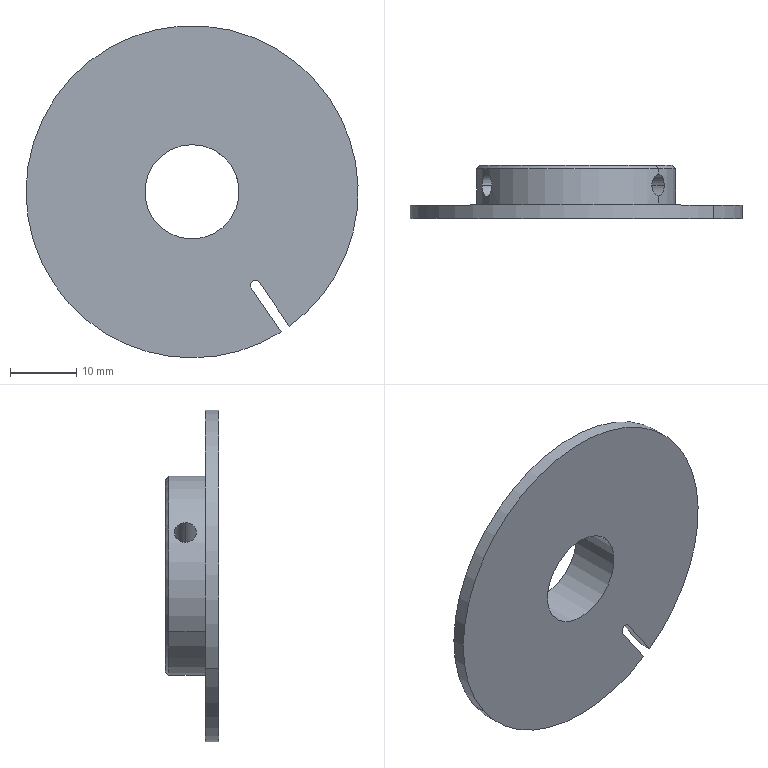Component | SolidWorks | H2020022-0437-1-2 | 1 solid | 19 faces | box 50 x 8 x 50 mm | volume 6728 mm3 | cylinder 12 | plane 5 | cone 2 | commonest cylinder face diameters 3.3 x4 50 x3 14.2 x2 30 x2 1.5 x1 | material 45#Steel
build123d program:
from build123d import *

# Parameters (mm, degrees)
SKETCH1_R           = 15
SKETCH1_R_2         = 7.1
BOSS_EXTRUDE1_DEPTH = 8
SKETCH3_W           = 1.65
SKETCH3_H           = 15
CIRPATTERN1_COUNT   = 2
CIRPATTERN1_ANGLE   = 120
CHAMFER2_SIZE       = 0.5
BOSS_EXTRUDE2_START = -2
SKETCH6_R           = 25
SKETCH6_R_2         = 15
BOSS_EXTRUDE2_DEPTH = 2
CUT_EXTRUDE1_DEPTH  = 37.249


with BuildPart() as part:
    # Sketch1 → Boss-Extrude1 (new body)
    with BuildSketch(Plane(origin=(0, 0, 0), x_dir=(1, 0, 0), z_dir=(0, 1, 0))):
        with Locations(Location((0, 0, 0), (0, 0, 270))):
            Circle(SKETCH1_R)
        with Locations(Location((0, 0, 0), (0, 0, 270))):
            Circle(SKETCH1_R_2, mode=Mode.SUBTRACT)
    extrude(amount=BOSS_EXTRUDE1_DEPTH)

    # Sketch3 → M4 Tapped Hole2 (revolve, cut)
    with BuildSketch(Plane(origin=(0, 3, 0), x_dir=(0, 1, 0), z_dir=(1, 0, 0))):
        with Locations((0.825, 7.5)):
            Rectangle(SKETCH3_W, SKETCH3_H)
    m4_tapped_hole2 = revolve(axis=Axis((0, 3, -6.35), (0, 0, 1)), mode=Mode.SUBTRACT)

    # CirPattern1: M4 Tapped Hole2 ×2 about axis
    cirpattern1_axis = Axis((0, 8, 0), (0, 1, 0))
    for i in range(1, CIRPATTERN1_COUNT):
        add(m4_tapped_hole2.rotate(cirpattern1_axis, i * CIRPATTERN1_ANGLE / (CIRPATTERN1_COUNT - 1)), mode=Mode.SUBTRACT)

    # Chamfer2
    chamfer2_edges = [part.edges().sort_by_distance(p)[0] for p in [
        (0, 0, -15),
    ]]
    chamfer(chamfer2_edges, length=CHAMFER2_SIZE)

    # Sketch6 → Boss-Extrude2 (add)
    with BuildSketch(Plane(origin=(0, 8, 0), x_dir=(1, 0, 0), z_dir=(0, 1, 0)).offset(BOSS_EXTRUDE2_START)):
        with Locations(Location((0, 0, 0), (0, 0, 270))):
            Circle(SKETCH6_R)
        with Locations(Location((0, 0, 0), (0, 0, 270))):
            Circle(SKETCH6_R_2, mode=Mode.SUBTRACT)
    extrude(amount=BOSS_EXTRUDE2_DEPTH)

    # Sketch7 → Cut-Extrude1 (cut, through all)
    with BuildSketch(Plane(origin=(0, 8, 0), x_dir=(1, 0, 0), z_dir=(0, 1, 0))):
        with BuildLine():
            Line((-25, 0.75), (-17, 0.75))
            ThreePointArc((-17, 0.75), (-16.25, 0), (-17, -0.75))
            Line((-17, -0.75), (-25, -0.75))
            ThreePointArc((-25, -0.75), (-25.75, 0), (-25, 0.75))
        make_face()
    extrude(amount=-CUT_EXTRUDE1_DEPTH, mode=Mode.SUBTRACT)


solid = part.part

# Placed as in the assembly
solid = solid.moved(Location((-30.964, 61.013, 280.197), (0, 55.863, 180)))
STEP:
#1=COLOUR_RGB('',0.7922,0.8196,0.9333);
#2=FILL_AREA_STYLE_COLOUR('',#1);
#3=FILL_AREA_STYLE('',(#2));
#4=SURFACE_STYLE_FILL_AREA(#3);
#5=SURFACE_SIDE_STYLE('',(#4));
#6=SURFACE_STYLE_USAGE(.BOTH.,#5);
#7=PRESENTATION_STYLE_ASSIGNMENT((#6));
#8=CARTESIAN_POINT('',(-0.4044,2.166,11.584));
#9=VERTEX_POINT('',#8);
#10=CARTESIAN_POINT('',(-2.034,2.166,10.479));
#11=VERTEX_POINT('',#10);
#12=CARTESIAN_POINT('',(-1.219,2.166,11.031));
#13=DIRECTION('',(0.,-1.,0.));
#14=DIRECTION('',(0.8277,0.,0.5612));
#15=AXIS2_PLACEMENT_3D('',#12,#13,#14);
#16=CIRCLE('',#15,0.9843);
#17=EDGE_CURVE('',#9,#11,#16,.T.);
#18=ORIENTED_EDGE('',*,*,#17,.T.);
#19=CARTESIAN_POINT('',(-2.034,2.087,10.479));
#20=VERTEX_POINT('',#19);
#21=CARTESIAN_POINT('',(-2.034,2.166,10.479));
#22=DIRECTION('',(0.,-1.,0.));
#23=VECTOR('',#22,39.37);
#24=LINE('',#21,#23);
#25=EDGE_CURVE('',#11,#20,#24,.T.);
#26=ORIENTED_EDGE('',*,*,#25,.T.);
#27=CARTESIAN_POINT('',(-0.4044,2.087,11.584));
#28=VERTEX_POINT('',#27);
#29=CARTESIAN_POINT('',(-1.219,2.087,11.031));
#30=DIRECTION('',(0.,-1.,0.));
#31=DIRECTION('',(0.8277,0.,0.5612));
#32=AXIS2_PLACEMENT_3D('',#29,#30,#31);
#33=CIRCLE('',#32,0.9843);
#34=EDGE_CURVE('',#28,#20,#33,.T.);
#35=ORIENTED_EDGE('',*,*,#34,.F.);
#36=CARTESIAN_POINT('',(-0.4044,2.166,11.584));
#37=DIRECTION('',(0.,-1.,0.));
#38=VECTOR('',#37,39.37);
#39=LINE('',#36,#38);
#40=EDGE_CURVE('',#9,#28,#39,.T.);
#41=ORIENTED_EDGE('',*,*,#40,.F.);
#42=EDGE_LOOP('',(#18,#26,#35,#41));
#43=FACE_OUTER_BOUND('',#42,.T.);
#44=CARTESIAN_POINT('',(-1.219,2.166,11.031));
#45=DIRECTION('',(0.,-1.,0.));
#46=DIRECTION('',(0.8277,0.,0.5612));
#47=AXIS2_PLACEMENT_3D('',#44,#45,#46);
#48=CYLINDRICAL_SURFACE('',#47,0.9843);
#49=ADVANCED_FACE('',(#43),#48,.T.);
#50=CARTESIAN_POINT('',(-0.6425,2.166,10.234));
#51=VERTEX_POINT('',#50);
#52=CARTESIAN_POINT('',(-1.219,2.166,11.031));
#53=DIRECTION('',(0.,-1.,0.));
#54=DIRECTION('',(0.8277,0.,0.5612));
#55=AXIS2_PLACEMENT_3D('',#52,#53,#54);
#56=CIRCLE('',#55,0.9843);
#57=EDGE_CURVE('',#51,#9,#56,.T.);
#58=ORIENTED_EDGE('',*,*,#57,.T.);
#59=ORIENTED_EDGE('',*,*,#40,.T.);
#60=CARTESIAN_POINT('',(-0.6425,2.087,10.234));
#61=VERTEX_POINT('',#60);
#62=CARTESIAN_POINT('',(-1.219,2.087,11.031));
#63=DIRECTION('',(0.,-1.,0.));
#64=DIRECTION('',(0.8277,0.,0.5612));
#65=AXIS2_PLACEMENT_3D('',#62,#63,#64);
#66=CIRCLE('',#65,0.9843);
#67=EDGE_CURVE('',#61,#28,#66,.T.);
#68=ORIENTED_EDGE('',*,*,#67,.F.);
#69=CARTESIAN_POINT('',(-0.6425,2.166,10.234));
#70=DIRECTION('',(0.,-1.,0.));
#71=VECTOR('',#70,39.37);
#72=LINE('',#69,#71);
#73=EDGE_CURVE('',#51,#61,#72,.T.);
#74=ORIENTED_EDGE('',*,*,#73,.F.);
#75=EDGE_LOOP('',(#58,#59,#68,#74));
#76=FACE_OUTER_BOUND('',#75,.T.);
#77=CARTESIAN_POINT('',(-1.219,2.166,11.031));
#78=DIRECTION('',(0.,-1.,0.));
#79=DIRECTION('',(0.8277,0.,0.5612));
#80=AXIS2_PLACEMENT_3D('',#77,#78,#79);
#81=CYLINDRICAL_SURFACE('',#80,0.9843);
#82=ADVANCED_FACE('',(#76),#81,.T.);
#83=CARTESIAN_POINT('',(-1.692,2.402,10.711));
#84=VERTEX_POINT('',#83);
#85=CARTESIAN_POINT('',(-0.7466,2.402,11.352));
#86=VERTEX_POINT('',#85);
#87=CARTESIAN_POINT('',(-1.219,2.402,11.031));
#88=DIRECTION('',(0.,1.,0.));
#89=DIRECTION('',(0.8277,0.,0.5612));
#90=AXIS2_PLACEMENT_3D('',#87,#88,#89);
#91=CIRCLE('',#90,0.5709);
#92=EDGE_CURVE('',#84,#86,#91,.T.);
#93=ORIENTED_EDGE('',*,*,#92,.F.);
#94=CARTESIAN_POINT('',(-1.708,2.382,10.7));
#95=VERTEX_POINT('',#94);
#96=CARTESIAN_POINT('',(-1.708,2.382,10.7));
#97=DIRECTION('',(-0.5853,-0.7071,-0.3968));
#98=VECTOR('',#97,39.37);
#99=LINE('',#96,#98);
#100=EDGE_CURVE('',#84,#95,#99,.T.);
#101=ORIENTED_EDGE('',*,*,#100,.T.);
#102=CARTESIAN_POINT('',(-0.7303,2.382,11.363));
#103=VERTEX_POINT('',#102);
#104=CARTESIAN_POINT('',(-1.219,2.382,11.031));
#105=DIRECTION('',(0.,-1.,0.));
#106=DIRECTION('',(0.8277,0.,0.5612));
#107=AXIS2_PLACEMENT_3D('',#104,#105,#106);
#108=CIRCLE('',#107,0.5906);
#109=EDGE_CURVE('',#103,#95,#108,.T.);
#110=ORIENTED_EDGE('',*,*,#109,.F.);
#111=CARTESIAN_POINT('',(-0.7303,2.382,11.363));
#112=DIRECTION('',(0.5853,-0.7071,0.3968));
#113=VECTOR('',#112,39.37);
#114=LINE('',#111,#113);
#115=EDGE_CURVE('',#86,#103,#114,.T.);
#116=ORIENTED_EDGE('',*,*,#115,.F.);
#117=EDGE_LOOP('',(#93,#101,#110,#116));
#118=FACE_OUTER_BOUND('',#117,.T.);
#119=CARTESIAN_POINT('',(-1.219,2.382,11.031));
#120=DIRECTION('',(0.,-1.,0.));
#121=DIRECTION('',(0.8277,0.,0.5612));
#122=AXIS2_PLACEMENT_3D('',#119,#120,#121);
#123=CONICAL_SURFACE('',#122,0.5906,0.7854);
#124=ADVANCED_FACE('',(#118),#123,.T.);
#125=CARTESIAN_POINT('',(-1.776,2.284,11.229));
#126=VERTEX_POINT('',#125);
#127=CARTESIAN_POINT('',(-1.719,2.284,11.346));
#128=VERTEX_POINT('',#127);
#129=CARTESIAN_POINT('',(-1.776,2.284,11.229));
#130=CARTESIAN_POINT('',(-1.776,2.292,11.229));
#131=CARTESIAN_POINT('',(-1.775,2.301,11.231));
#132=CARTESIAN_POINT('',(-1.773,2.317,11.237));
#133=CARTESIAN_POINT('',(-1.771,2.324,11.241));
#134=CARTESIAN_POINT('',(-1.768,2.333,11.25));
#135=CARTESIAN_POINT('',(-1.767,2.336,11.253));
#136=CARTESIAN_POINT('',(-1.764,2.34,11.259));
#137=CARTESIAN_POINT('',(-1.762,2.342,11.263));
#138=CARTESIAN_POINT('',(-1.759,2.346,11.27));
#139=CARTESIAN_POINT('',(-1.758,2.347,11.274));
#140=CARTESIAN_POINT('',(-1.754,2.348,11.281));
#141=CARTESIAN_POINT('',(-1.752,2.349,11.285));
#142=CARTESIAN_POINT('',(-1.749,2.349,11.293));
#143=CARTESIAN_POINT('',(-1.747,2.349,11.297));
#144=CARTESIAN_POINT('',(-1.743,2.347,11.304));
#145=CARTESIAN_POINT('',(-1.741,2.346,11.308));
#146=CARTESIAN_POINT('',(-1.737,2.342,11.315));
#147=CARTESIAN_POINT('',(-1.735,2.34,11.318));
#148=CARTESIAN_POINT('',(-1.732,2.336,11.324));
#149=CARTESIAN_POINT('',(-1.73,2.333,11.327));
#150=CARTESIAN_POINT('',(-1.726,2.324,11.335));
#151=CARTESIAN_POINT('',(-1.723,2.317,11.339));
#152=CARTESIAN_POINT('',(-1.72,2.301,11.344));
#153=CARTESIAN_POINT('',(-1.719,2.293,11.346));
#154=CARTESIAN_POINT('',(-1.719,2.284,11.346));
#155=B_SPLINE_CURVE_WITH_KNOTS('',3,(#129,#130,#131,#132,#133,#134,#135,#136,#137,#138,#139,#140,#141,#142,#143,#144,#145,#146,#147,#148,#149,#150,#151,#152,#153,#154),.UNSPECIFIED.,.F.,.F.,(4,2,2,2,2,2,2,2,2,2,2,2,4),(0.005163,0.005808,0.006453,0.006775,0.007098,0.007421,0.007743,0.008066,0.008388,0.008711,0.009034,0.009679,0.01032),.UNSPECIFIED.);
#156=EDGE_CURVE('',#126,#128,#155,.T.);
#157=ORIENTED_EDGE('',*,*,#156,.F.);
#158=CARTESIAN_POINT('',(-1.492,2.284,11.092));
#159=VERTEX_POINT('',#158);
#160=CARTESIAN_POINT('',(-1.247,2.284,10.973));
#161=DIRECTION('',(0.8998,0.,-0.4362));
#162=VECTOR('',#161,39.37);
#163=LINE('',#160,#162);
#164=EDGE_CURVE('',#126,#159,#163,.T.);
#165=ORIENTED_EDGE('',*,*,#164,.T.);
#166=CARTESIAN_POINT('',(-1.435,2.284,11.208));
#167=VERTEX_POINT('',#166);
#168=CARTESIAN_POINT('',(-1.492,2.284,11.092));
#169=CARTESIAN_POINT('',(-1.492,2.292,11.092));
#170=CARTESIAN_POINT('',(-1.492,2.301,11.093));
#171=CARTESIAN_POINT('',(-1.491,2.313,11.098));
#172=CARTESIAN_POINT('',(-1.49,2.317,11.1));
#173=CARTESIAN_POINT('',(-1.489,2.324,11.105));
#174=CARTESIAN_POINT('',(-1.488,2.327,11.107));
#175=CARTESIAN_POINT('',(-1.486,2.333,11.113));
#176=CARTESIAN_POINT('',(-1.485,2.336,11.116));
#177=CARTESIAN_POINT('',(-1.483,2.34,11.123));
#178=CARTESIAN_POINT('',(-1.482,2.342,11.127));
#179=CARTESIAN_POINT('',(-1.478,2.347,11.138));
#180=CARTESIAN_POINT('',(-1.474,2.349,11.146));
#181=CARTESIAN_POINT('',(-1.469,2.349,11.157));
#182=CARTESIAN_POINT('',(-1.467,2.349,11.161));
#183=CARTESIAN_POINT('',(-1.463,2.347,11.168));
#184=CARTESIAN_POINT('',(-1.461,2.346,11.172));
#185=CARTESIAN_POINT('',(-1.455,2.341,11.182));
#186=CARTESIAN_POINT('',(-1.451,2.336,11.188));
#187=CARTESIAN_POINT('',(-1.444,2.324,11.198));
#188=CARTESIAN_POINT('',(-1.441,2.317,11.202));
#189=CARTESIAN_POINT('',(-1.438,2.305,11.206));
#190=CARTESIAN_POINT('',(-1.437,2.301,11.207));
#191=CARTESIAN_POINT('',(-1.436,2.293,11.208));
#192=CARTESIAN_POINT('',(-1.435,2.288,11.208));
#193=CARTESIAN_POINT('',(-1.435,2.284,11.208));
#194=B_SPLINE_CURVE_WITH_KNOTS('',3,(#168,#169,#170,#171,#172,#173,#174,#175,#176,#177,#178,#179,#180,#181,#182,#183,#184,#185,#186,#187,#188,#189,#190,#191,#192,#193),.UNSPECIFIED.,.F.,.F.,(4,2,2,2,2,2,2,2,2,2,2,2,4),(0.005176,0.005823,0.006147,0.00647,0.006794,0.007117,0.007764,0.008087,0.008411,0.009058,0.009704,0.01003,0.01035),.UNSPECIFIED.);
#195=EDGE_CURVE('',#159,#167,#194,.T.);
#196=ORIENTED_EDGE('',*,*,#195,.T.);
#197=CARTESIAN_POINT('',(-1.191,2.284,11.09));
#198=DIRECTION('',(0.8998,0.,-0.4362));
#199=VECTOR('',#198,39.37);
#200=LINE('',#197,#199);
#201=EDGE_CURVE('',#128,#167,#200,.T.);
#202=ORIENTED_EDGE('',*,*,#201,.F.);
#203=EDGE_LOOP('',(#157,#165,#196,#202));
#204=FACE_OUTER_BOUND('',#203,.T.);
#205=CARTESIAN_POINT('',(-1.219,2.284,11.031));
#206=DIRECTION('',(0.8998,0.,-0.4362));
#207=DIRECTION('',(0.4362,0.,0.8998));
#208=AXIS2_PLACEMENT_3D('',#205,#206,#207);
#209=CYLINDRICAL_SURFACE('',#208,0.06496);
#210=ADVANCED_FACE('',(#204),#209,.F.);
#211=CARTESIAN_POINT('',(-0.7697,2.284,11.415));
#212=VERTEX_POINT('',#211);
#213=CARTESIAN_POINT('',(-0.7303,2.349,11.363));
#214=VERTEX_POINT('',#213);
#215=CARTESIAN_POINT('',(-0.7697,2.284,11.415));
#216=CARTESIAN_POINT('',(-0.7697,2.288,11.415));
#217=CARTESIAN_POINT('',(-0.7694,2.292,11.414));
#218=CARTESIAN_POINT('',(-0.7683,2.301,11.413));
#219=CARTESIAN_POINT('',(-0.7675,2.305,11.412));
#220=CARTESIAN_POINT('',(-0.7654,2.313,11.409));
#221=CARTESIAN_POINT('',(-0.7641,2.316,11.408));
#222=CARTESIAN_POINT('',(-0.7611,2.324,11.404));
#223=CARTESIAN_POINT('',(-0.7594,2.327,11.402));
#224=CARTESIAN_POINT('',(-0.7538,2.336,11.395));
#225=CARTESIAN_POINT('',(-0.7493,2.341,11.389));
#226=CARTESIAN_POINT('',(-0.74,2.347,11.377));
#227=CARTESIAN_POINT('',(-0.7351,2.349,11.37));
#228=CARTESIAN_POINT('',(-0.7303,2.349,11.363));
#229=B_SPLINE_CURVE_WITH_KNOTS('',3,(#215,#216,#217,#218,#219,#220,#221,#222,#223,#224,#225,#226,#227,#228),.UNSPECIFIED.,.F.,.F.,(4,2,2,2,2,2,4),(0.007744,0.008067,0.008389,0.008712,0.009034,0.009679,0.01032),.UNSPECIFIED.);
#230=EDGE_CURVE('',#212,#214,#229,.T.);
#231=ORIENTED_EDGE('',*,*,#230,.F.);
#232=CARTESIAN_POINT('',(-1.03,2.284,11.238));
#233=VERTEX_POINT('',#232);
#234=CARTESIAN_POINT('',(-1.256,2.284,11.085));
#235=DIRECTION('',(-0.8277,0.,-0.5612));
#236=VECTOR('',#235,39.37);
#237=LINE('',#234,#236);
#238=EDGE_CURVE('',#212,#233,#237,.T.);
#239=ORIENTED_EDGE('',*,*,#238,.T.);
#240=CARTESIAN_POINT('',(-0.9877,2.349,11.188));
#241=VERTEX_POINT('',#240);
#242=CARTESIAN_POINT('',(-1.03,2.284,11.238));
#243=CARTESIAN_POINT('',(-1.03,2.292,11.238));
#244=CARTESIAN_POINT('',(-1.029,2.301,11.237));
#245=CARTESIAN_POINT('',(-1.026,2.313,11.233));
#246=CARTESIAN_POINT('',(-1.024,2.317,11.232));
#247=CARTESIAN_POINT('',(-1.021,2.324,11.228));
#248=CARTESIAN_POINT('',(-1.019,2.327,11.226));
#249=CARTESIAN_POINT('',(-1.015,2.333,11.222));
#250=CARTESIAN_POINT('',(-1.012,2.336,11.219));
#251=CARTESIAN_POINT('',(-1.008,2.34,11.214));
#252=CARTESIAN_POINT('',(-1.005,2.342,11.211));
#253=CARTESIAN_POINT('',(-0.9976,2.347,11.202));
#254=CARTESIAN_POINT('',(-0.9925,2.349,11.195));
#255=CARTESIAN_POINT('',(-0.9877,2.349,11.188));
#256=B_SPLINE_CURVE_WITH_KNOTS('',3,(#242,#243,#244,#245,#246,#247,#248,#249,#250,#251,#252,#253,#254,#255),.UNSPECIFIED.,.F.,.F.,(4,2,2,2,2,2,4),(0.005176,0.005823,0.006147,0.00647,0.006794,0.007117,0.007764),.UNSPECIFIED.);
#257=EDGE_CURVE('',#233,#241,#256,.T.);
#258=ORIENTED_EDGE('',*,*,#257,.T.);
#259=CARTESIAN_POINT('',(-0.9576,2.284,11.13));
#260=VERTEX_POINT('',#259);
#261=CARTESIAN_POINT('',(-0.9877,2.349,11.188));
#262=CARTESIAN_POINT('',(-0.9853,2.349,11.185));
#263=CARTESIAN_POINT('',(-0.983,2.349,11.181));
#264=CARTESIAN_POINT('',(-0.9786,2.347,11.174));
#265=CARTESIAN_POINT('',(-0.9766,2.346,11.17));
#266=CARTESIAN_POINT('',(-0.9708,2.341,11.16));
#267=CARTESIAN_POINT('',(-0.9676,2.336,11.154));
#268=CARTESIAN_POINT('',(-0.9625,2.324,11.143));
#269=CARTESIAN_POINT('',(-0.9607,2.317,11.138));
#270=CARTESIAN_POINT('',(-0.9588,2.305,11.133));
#271=CARTESIAN_POINT('',(-0.9583,2.301,11.132));
#272=CARTESIAN_POINT('',(-0.9577,2.293,11.131));
#273=CARTESIAN_POINT('',(-0.9576,2.288,11.13));
#274=CARTESIAN_POINT('',(-0.9576,2.284,11.13));
#275=B_SPLINE_CURVE_WITH_KNOTS('',3,(#261,#262,#263,#264,#265,#266,#267,#268,#269,#270,#271,#272,#273,#274),.UNSPECIFIED.,.F.,.F.,(4,2,2,2,2,2,4),(0.007764,0.008088,0.008411,0.009058,0.009705,0.01003,0.01035),.UNSPECIFIED.);
#276=EDGE_CURVE('',#241,#260,#275,.T.);
#277=ORIENTED_EDGE('',*,*,#276,.T.);
#278=CARTESIAN_POINT('',(-0.6968,2.284,11.307));
#279=VERTEX_POINT('',#278);
#280=CARTESIAN_POINT('',(-1.183,2.284,10.978));
#281=DIRECTION('',(-0.8277,0.,-0.5612));
#282=VECTOR('',#281,39.37);
#283=LINE('',#280,#282);
#284=EDGE_CURVE('',#279,#260,#283,.T.);
#285=ORIENTED_EDGE('',*,*,#284,.F.);
#286=CARTESIAN_POINT('',(-0.7303,2.349,11.363));
#287=CARTESIAN_POINT('',(-0.7279,2.349,11.359));
#288=CARTESIAN_POINT('',(-0.7255,2.349,11.356));
#289=CARTESIAN_POINT('',(-0.721,2.347,11.349));
#290=CARTESIAN_POINT('',(-0.7188,2.346,11.345));
#291=CARTESIAN_POINT('',(-0.7147,2.342,11.339));
#292=CARTESIAN_POINT('',(-0.7127,2.34,11.335));
#293=CARTESIAN_POINT('',(-0.7091,2.336,11.329));
#294=CARTESIAN_POINT('',(-0.7074,2.333,11.326));
#295=CARTESIAN_POINT('',(-0.703,2.324,11.319));
#296=CARTESIAN_POINT('',(-0.7007,2.317,11.314));
#297=CARTESIAN_POINT('',(-0.6976,2.301,11.309));
#298=CARTESIAN_POINT('',(-0.6968,2.292,11.307));
#299=CARTESIAN_POINT('',(-0.6968,2.284,11.307));
#300=B_SPLINE_CURVE_WITH_KNOTS('',3,(#286,#287,#288,#289,#290,#291,#292,#293,#294,#295,#296,#297,#298,#299),.UNSPECIFIED.,.F.,.F.,(4,2,2,2,2,2,4),(0.,0.0003227,0.0006455,0.0009682,0.001291,0.001936,0.002582),.UNSPECIFIED.);
#301=EDGE_CURVE('',#214,#279,#300,.T.);
#302=ORIENTED_EDGE('',*,*,#301,.F.);
#303=EDGE_LOOP('',(#231,#239,#258,#277,#285,#302));
#304=FACE_OUTER_BOUND('',#303,.T.);
#305=CARTESIAN_POINT('',(-1.219,2.284,11.031));
#306=DIRECTION('',(-0.8277,0.,-0.5612));
#307=DIRECTION('',(0.5612,0.,-0.8277));
#308=AXIS2_PLACEMENT_3D('',#305,#306,#307);
#309=CYLINDRICAL_SURFACE('',#308,0.06496);
#310=ADVANCED_FACE('',(#304),#309,.F.);
#311=CARTESIAN_POINT('',(-1.45,2.087,10.875));
#312=VERTEX_POINT('',#311);
#313=CARTESIAN_POINT('',(-0.9877,2.087,11.188));
#314=VERTEX_POINT('',#313);
#315=CARTESIAN_POINT('',(-1.219,2.087,11.031));
#316=DIRECTION('',(0.,-1.,0.));
#317=DIRECTION('',(0.8277,0.,0.5612));
#318=AXIS2_PLACEMENT_3D('',#315,#316,#317);
#319=CIRCLE('',#318,0.2795);
#320=EDGE_CURVE('',#312,#314,#319,.T.);
#321=ORIENTED_EDGE('',*,*,#320,.T.);
#322=CARTESIAN_POINT('',(-0.9877,2.219,11.188));
#323=VERTEX_POINT('',#322);
#324=CARTESIAN_POINT('',(-0.9877,2.087,11.188));
#325=DIRECTION('',(0.,1.,0.));
#326=VECTOR('',#325,39.37);
#327=LINE('',#324,#326);
#328=EDGE_CURVE('',#314,#323,#327,.T.);
#329=ORIENTED_EDGE('',*,*,#328,.T.);
#330=CARTESIAN_POINT('',(-0.9576,2.284,11.13));
#331=CARTESIAN_POINT('',(-0.9576,2.28,11.13));
#332=CARTESIAN_POINT('',(-0.9577,2.275,11.131));
#333=CARTESIAN_POINT('',(-0.9583,2.267,11.132));
#334=CARTESIAN_POINT('',(-0.9588,2.263,11.133));
#335=CARTESIAN_POINT('',(-0.96,2.255,11.136));
#336=CARTESIAN_POINT('',(-0.9608,2.251,11.138));
#337=CARTESIAN_POINT('',(-0.9627,2.244,11.143));
#338=CARTESIAN_POINT('',(-0.9638,2.241,11.145));
#339=CARTESIAN_POINT('',(-0.9676,2.232,11.154));
#340=CARTESIAN_POINT('',(-0.9708,2.227,11.16));
#341=CARTESIAN_POINT('',(-0.9785,2.221,11.174));
#342=CARTESIAN_POINT('',(-0.9829,2.219,11.181));
#343=CARTESIAN_POINT('',(-0.9877,2.219,11.188));
#344=B_SPLINE_CURVE_WITH_KNOTS('',3,(#330,#331,#332,#333,#334,#335,#336,#337,#338,#339,#340,#341,#342,#343),.UNSPECIFIED.,.F.,.F.,(4,2,2,2,2,2,4),(0.,0.0003236,0.0006472,0.0009708,0.001294,0.001942,0.002589),.UNSPECIFIED.);
#345=EDGE_CURVE('',#260,#323,#344,.T.);
#346=ORIENTED_EDGE('',*,*,#345,.F.);
#347=ORIENTED_EDGE('',*,*,#276,.F.);
#348=CARTESIAN_POINT('',(-0.9877,2.402,11.188));
#349=VERTEX_POINT('',#348);
#350=CARTESIAN_POINT('',(-0.9877,2.087,11.188));
#351=DIRECTION('',(0.,1.,0.));
#352=VECTOR('',#351,39.37);
#353=LINE('',#350,#352);
#354=EDGE_CURVE('',#241,#349,#353,.T.);
#355=ORIENTED_EDGE('',*,*,#354,.T.);
#356=CARTESIAN_POINT('',(-1.45,2.402,10.875));
#357=VERTEX_POINT('',#356);
#358=CARTESIAN_POINT('',(-1.219,2.402,11.031));
#359=DIRECTION('',(0.,-1.,0.));
#360=DIRECTION('',(0.8277,0.,0.5612));
#361=AXIS2_PLACEMENT_3D('',#358,#359,#360);
#362=CIRCLE('',#361,0.2795);
#363=EDGE_CURVE('',#357,#349,#362,.T.);
#364=ORIENTED_EDGE('',*,*,#363,.F.);
#365=CARTESIAN_POINT('',(-1.45,2.087,10.875));
#366=DIRECTION('',(0.,1.,0.));
#367=VECTOR('',#366,39.37);
#368=LINE('',#365,#367);
#369=EDGE_CURVE('',#312,#357,#368,.T.);
#370=ORIENTED_EDGE('',*,*,#369,.F.);
#371=EDGE_LOOP('',(#321,#329,#346,#347,#355,#364,#370));
#372=FACE_OUTER_BOUND('',#371,.T.);
#373=CARTESIAN_POINT('',(-1.219,2.087,11.031));
#374=DIRECTION('',(0.,1.,0.));
#375=DIRECTION('',(-0.8277,0.,-0.5612));
#376=AXIS2_PLACEMENT_3D('',#373,#374,#375);
#377=CYLINDRICAL_SURFACE('',#376,0.2795);
#378=ADVANCED_FACE('',(#372),#377,.F.);
#379=CARTESIAN_POINT('',(-1.719,2.284,11.346));
#380=CARTESIAN_POINT('',(-1.719,2.28,11.346));
#381=CARTESIAN_POINT('',(-1.719,2.275,11.346));
#382=CARTESIAN_POINT('',(-1.72,2.267,11.344));
#383=CARTESIAN_POINT('',(-1.721,2.263,11.343));
#384=CARTESIAN_POINT('',(-1.722,2.255,11.34));
#385=CARTESIAN_POINT('',(-1.723,2.251,11.339));
#386=CARTESIAN_POINT('',(-1.726,2.244,11.334));
#387=CARTESIAN_POINT('',(-1.727,2.241,11.332));
#388=CARTESIAN_POINT('',(-1.732,2.232,11.324));
#389=CARTESIAN_POINT('',(-1.735,2.227,11.318));
#390=CARTESIAN_POINT('',(-1.743,2.221,11.304));
#391=CARTESIAN_POINT('',(-1.747,2.219,11.297));
#392=CARTESIAN_POINT('',(-1.752,2.219,11.285));
#393=CARTESIAN_POINT('',(-1.754,2.219,11.281));
#394=CARTESIAN_POINT('',(-1.758,2.221,11.274));
#395=CARTESIAN_POINT('',(-1.759,2.222,11.27));
#396=CARTESIAN_POINT('',(-1.762,2.226,11.263));
#397=CARTESIAN_POINT('',(-1.764,2.228,11.259));
#398=CARTESIAN_POINT('',(-1.767,2.232,11.253));
#399=CARTESIAN_POINT('',(-1.768,2.235,11.25));
#400=CARTESIAN_POINT('',(-1.77,2.241,11.244));
#401=CARTESIAN_POINT('',(-1.771,2.244,11.242));
#402=CARTESIAN_POINT('',(-1.773,2.251,11.237));
#403=CARTESIAN_POINT('',(-1.773,2.255,11.235));
#404=CARTESIAN_POINT('',(-1.774,2.263,11.232));
#405=CARTESIAN_POINT('',(-1.775,2.267,11.231));
#406=CARTESIAN_POINT('',(-1.775,2.275,11.229));
#407=CARTESIAN_POINT('',(-1.776,2.28,11.229));
#408=CARTESIAN_POINT('',(-1.776,2.284,11.229));
#409=B_SPLINE_CURVE_WITH_KNOTS('',3,(#379,#380,#381,#382,#383,#384,#385,#386,#387,#388,#389,#390,#391,#392,#393,#394,#395,#396,#397,#398,#399,#400,#401,#402,#403,#404,#405,#406,#407,#408),.UNSPECIFIED.,.F.,.F.,(4,2,2,2,2,2,2,2,2,2,2,2,2,2,4),(0.,0.0003227,0.0006453,0.000968,0.001291,0.001936,0.002581,0.002904,0.003227,0.003549,0.003872,0.004195,0.004517,0.00484,0.005163),.UNSPECIFIED.);
#410=EDGE_CURVE('',#128,#126,#409,.T.);
#411=ORIENTED_EDGE('',*,*,#410,.T.);
#412=ORIENTED_EDGE('',*,*,#156,.T.);
#413=EDGE_LOOP('',(#411,#412));
#414=FACE_BOUND('',#413,.T.);
#415=CARTESIAN_POINT('',(-0.7303,2.166,11.363));
#416=VERTEX_POINT('',#415);
#417=CARTESIAN_POINT('',(-1.708,2.166,10.7));
#418=VERTEX_POINT('',#417);
#419=CARTESIAN_POINT('',(-1.219,2.166,11.031));
#420=DIRECTION('',(0.,-1.,0.));
#421=DIRECTION('',(0.8277,0.,0.5612));
#422=AXIS2_PLACEMENT_3D('',#419,#420,#421);
#423=CIRCLE('',#422,0.5906);
#424=EDGE_CURVE('',#416,#418,#423,.T.);
#425=ORIENTED_EDGE('',*,*,#424,.F.);
#426=CARTESIAN_POINT('',(-0.7303,2.219,11.363));
#427=VERTEX_POINT('',#426);
#428=CARTESIAN_POINT('',(-0.7303,2.087,11.363));
#429=DIRECTION('',(0.,1.,0.));
#430=VECTOR('',#429,39.37);
#431=LINE('',#428,#430);
#432=EDGE_CURVE('',#416,#427,#431,.T.);
#433=ORIENTED_EDGE('',*,*,#432,.T.);
#434=CARTESIAN_POINT('',(-0.7303,2.219,11.363));
#435=CARTESIAN_POINT('',(-0.735,2.219,11.37));
#436=CARTESIAN_POINT('',(-0.74,2.221,11.377));
#437=CARTESIAN_POINT('',(-0.7493,2.227,11.389));
#438=CARTESIAN_POINT('',(-0.7538,2.232,11.395));
#439=CARTESIAN_POINT('',(-0.7594,2.241,11.402));
#440=CARTESIAN_POINT('',(-0.7611,2.244,11.404));
#441=CARTESIAN_POINT('',(-0.7641,2.251,11.408));
#442=CARTESIAN_POINT('',(-0.7654,2.255,11.409));
#443=CARTESIAN_POINT('',(-0.7675,2.263,11.412));
#444=CARTESIAN_POINT('',(-0.7683,2.267,11.413));
#445=CARTESIAN_POINT('',(-0.7694,2.275,11.414));
#446=CARTESIAN_POINT('',(-0.7697,2.28,11.415));
#447=CARTESIAN_POINT('',(-0.7697,2.284,11.415));
#448=B_SPLINE_CURVE_WITH_KNOTS('',3,(#434,#435,#436,#437,#438,#439,#440,#441,#442,#443,#444,#445,#446,#447),.UNSPECIFIED.,.F.,.F.,(4,2,2,2,2,2,4),(0.005163,0.005808,0.006453,0.006776,0.007099,0.007422,0.007744),.UNSPECIFIED.);
#449=EDGE_CURVE('',#427,#212,#448,.T.);
#450=ORIENTED_EDGE('',*,*,#449,.T.);
#451=ORIENTED_EDGE('',*,*,#230,.T.);
#452=CARTESIAN_POINT('',(-0.7303,2.087,11.363));
#453=DIRECTION('',(0.,1.,0.));
#454=VECTOR('',#453,39.37);
#455=LINE('',#452,#454);
#456=EDGE_CURVE('',#214,#103,#455,.T.);
#457=ORIENTED_EDGE('',*,*,#456,.T.);
#458=ORIENTED_EDGE('',*,*,#109,.T.);
#459=CARTESIAN_POINT('',(-1.708,2.087,10.7));
#460=DIRECTION('',(0.,1.,0.));
#461=VECTOR('',#460,39.37);
#462=LINE('',#459,#461);
#463=EDGE_CURVE('',#418,#95,#462,.T.);
#464=ORIENTED_EDGE('',*,*,#463,.F.);
#465=EDGE_LOOP('',(#425,#433,#450,#451,#457,#458,#464));
#466=FACE_OUTER_BOUND('',#465,.T.);
#467=CARTESIAN_POINT('',(-1.219,2.087,11.031));
#468=DIRECTION('',(0.,1.,0.));
#469=DIRECTION('',(-0.8277,0.,-0.5612));
#470=AXIS2_PLACEMENT_3D('',#467,#468,#469);
#471=CYLINDRICAL_SURFACE('',#470,0.5906);
#472=ADVANCED_FACE('',(#414,#466),#471,.T.);
#473=ORIENTED_EDGE('',*,*,#432,.F.);
#474=CARTESIAN_POINT('',(-1.219,2.166,11.031));
#475=DIRECTION('',(0.,-1.,0.));
#476=DIRECTION('',(0.8277,0.,0.5612));
#477=AXIS2_PLACEMENT_3D('',#474,#475,#476);
#478=CIRCLE('',#477,0.5906);
#479=EDGE_CURVE('',#418,#416,#478,.T.);
#480=ORIENTED_EDGE('',*,*,#479,.F.);
#481=ORIENTED_EDGE('',*,*,#463,.T.);
#482=CARTESIAN_POINT('',(-1.219,2.382,11.031));
#483=DIRECTION('',(0.,-1.,0.));
#484=DIRECTION('',(0.8277,0.,0.5612));
#485=AXIS2_PLACEMENT_3D('',#482,#483,#484);
#486=CIRCLE('',#485,0.5906);
#487=EDGE_CURVE('',#95,#103,#486,.T.);
#488=ORIENTED_EDGE('',*,*,#487,.T.);
#489=ORIENTED_EDGE('',*,*,#456,.F.);
#490=ORIENTED_EDGE('',*,*,#301,.T.);
#491=CARTESIAN_POINT('',(-0.6968,2.284,11.307));
#492=CARTESIAN_POINT('',(-0.6968,2.28,11.307));
#493=CARTESIAN_POINT('',(-0.697,2.275,11.307));
#494=CARTESIAN_POINT('',(-0.6978,2.267,11.309));
#495=CARTESIAN_POINT('',(-0.6983,2.263,11.31));
#496=CARTESIAN_POINT('',(-0.6999,2.255,11.313));
#497=CARTESIAN_POINT('',(-0.7009,2.251,11.315));
#498=CARTESIAN_POINT('',(-0.7031,2.244,11.319));
#499=CARTESIAN_POINT('',(-0.7045,2.241,11.321));
#500=CARTESIAN_POINT('',(-0.7075,2.235,11.326));
#501=CARTESIAN_POINT('',(-0.7091,2.232,11.329));
#502=CARTESIAN_POINT('',(-0.7127,2.228,11.335));
#503=CARTESIAN_POINT('',(-0.7147,2.226,11.339));
#504=CARTESIAN_POINT('',(-0.7188,2.222,11.345));
#505=CARTESIAN_POINT('',(-0.721,2.221,11.349));
#506=CARTESIAN_POINT('',(-0.7255,2.219,11.356));
#507=CARTESIAN_POINT('',(-0.7279,2.219,11.359));
#508=CARTESIAN_POINT('',(-0.7303,2.219,11.363));
#509=B_SPLINE_CURVE_WITH_KNOTS('',3,(#491,#492,#493,#494,#495,#496,#497,#498,#499,#500,#501,#502,#503,#504,#505,#506,#507,#508),.UNSPECIFIED.,.F.,.F.,(4,2,2,2,2,2,2,2,4),(0.002582,0.002904,0.003227,0.00355,0.003872,0.004195,0.004517,0.00484,0.005163),.UNSPECIFIED.);
#510=EDGE_CURVE('',#279,#427,#509,.T.);
#511=ORIENTED_EDGE('',*,*,#510,.T.);
#512=EDGE_LOOP('',(#473,#480,#481,#488,#489,#490,#511));
#513=FACE_OUTER_BOUND('',#512,.T.);
#514=CARTESIAN_POINT('',(-1.219,2.087,11.031));
#515=DIRECTION('',(0.,1.,0.));
#516=DIRECTION('',(-0.8277,0.,-0.5612));
#517=AXIS2_PLACEMENT_3D('',#514,#515,#516);
#518=CYLINDRICAL_SURFACE('',#517,0.5906);
#519=ADVANCED_FACE('',(#513),#518,.T.);
#520=CARTESIAN_POINT('',(-0.8679,2.087,10.461));
#521=VERTEX_POINT('',#520);
#522=CARTESIAN_POINT('',(-0.6914,2.087,10.2));
#523=VERTEX_POINT('',#522);
#524=CARTESIAN_POINT('',(-0.6912,2.087,10.2));
#525=DIRECTION('',(0.5612,0.,-0.8277));
#526=VECTOR('',#525,39.37);
#527=LINE('',#524,#526);
#528=EDGE_CURVE('',#521,#523,#527,.T.);
#529=ORIENTED_EDGE('',*,*,#528,.F.);
#530=CARTESIAN_POINT('',(-0.819,2.087,10.494));
#531=VERTEX_POINT('',#530);
#532=CARTESIAN_POINT('',(-0.8435,2.087,10.477));
#533=DIRECTION('',(0.,-1.,0.));
#534=DIRECTION('',(0.8277,0.,0.5612));
#535=AXIS2_PLACEMENT_3D('',#532,#533,#534);
#536=CIRCLE('',#535,0.02953);
#537=EDGE_CURVE('',#531,#521,#536,.T.);
#538=ORIENTED_EDGE('',*,*,#537,.F.);
#539=CARTESIAN_POINT('',(-0.6423,2.087,10.233));
#540=DIRECTION('',(-0.5612,0.,0.8277));
#541=VECTOR('',#540,39.37);
#542=LINE('',#539,#541);
#543=EDGE_CURVE('',#61,#531,#542,.T.);
#544=ORIENTED_EDGE('',*,*,#543,.F.);
#545=ORIENTED_EDGE('',*,*,#67,.T.);
#546=ORIENTED_EDGE('',*,*,#34,.T.);
#547=CARTESIAN_POINT('',(-1.219,2.087,11.031));
#548=DIRECTION('',(0.,-1.,0.));
#549=DIRECTION('',(0.8277,0.,0.5612));
#550=AXIS2_PLACEMENT_3D('',#547,#548,#549);
#551=CIRCLE('',#550,0.9843);
#552=EDGE_CURVE('',#20,#523,#551,.T.);
#553=ORIENTED_EDGE('',*,*,#552,.T.);
#554=EDGE_LOOP('',(#529,#538,#544,#545,#546,#553));
#555=FACE_OUTER_BOUND('',#554,.T.);
#556=ORIENTED_EDGE('',*,*,#320,.F.);
#557=CARTESIAN_POINT('',(-1.219,2.087,11.031));
#558=DIRECTION('',(0.,-1.,0.));
#559=DIRECTION('',(0.8277,0.,0.5612));
#560=AXIS2_PLACEMENT_3D('',#557,#558,#559);
#561=CIRCLE('',#560,0.2795);
#562=EDGE_CURVE('',#314,#312,#561,.T.);
#563=ORIENTED_EDGE('',*,*,#562,.F.);
#564=EDGE_LOOP('',(#556,#563));
#565=FACE_BOUND('',#564,.T.);
#566=CARTESIAN_POINT('',(-1.219,2.087,11.031));
#567=DIRECTION('',(0.,-1.,0.));
#568=DIRECTION('',(0.8277,0.,0.5612));
#569=AXIS2_PLACEMENT_3D('',#566,#567,#568);
#570=PLANE('',#569);
#571=ADVANCED_FACE('',(#555,#565),#570,.T.);
#572=CARTESIAN_POINT('',(-1.219,2.402,11.031));
#573=DIRECTION('',(0.,1.,0.));
#574=DIRECTION('',(0.8277,0.,0.5612));
#575=AXIS2_PLACEMENT_3D('',#572,#573,#574);
#576=CIRCLE('',#575,0.5709);
#577=EDGE_CURVE('',#86,#84,#576,.T.);
#578=ORIENTED_EDGE('',*,*,#577,.T.);
#579=ORIENTED_EDGE('',*,*,#92,.T.);
#580=EDGE_LOOP('',(#578,#579));
#581=FACE_OUTER_BOUND('',#580,.T.);
#582=ORIENTED_EDGE('',*,*,#363,.T.);
#583=CARTESIAN_POINT('',(-1.219,2.402,11.031));
#584=DIRECTION('',(0.,-1.,0.));
#585=DIRECTION('',(0.8277,0.,0.5612));
#586=AXIS2_PLACEMENT_3D('',#583,#584,#585);
#587=CIRCLE('',#586,0.2795);
#588=EDGE_CURVE('',#349,#357,#587,.T.);
#589=ORIENTED_EDGE('',*,*,#588,.T.);
#590=EDGE_LOOP('',(#582,#589));
#591=FACE_BOUND('',#590,.T.);
#592=CARTESIAN_POINT('',(-1.219,2.402,11.031));
#593=DIRECTION('',(0.,-1.,0.));
#594=DIRECTION('',(0.8277,0.,0.5612));
#595=AXIS2_PLACEMENT_3D('',#592,#593,#594);
#596=PLANE('',#595);
#597=ADVANCED_FACE('',(#581,#591),#596,.F.);
#598=ORIENTED_EDGE('',*,*,#328,.F.);
#599=ORIENTED_EDGE('',*,*,#562,.T.);
#600=ORIENTED_EDGE('',*,*,#369,.T.);
#601=ORIENTED_EDGE('',*,*,#588,.F.);
#602=ORIENTED_EDGE('',*,*,#354,.F.);
#603=ORIENTED_EDGE('',*,*,#257,.F.);
#604=CARTESIAN_POINT('',(-0.9877,2.219,11.188));
#605=CARTESIAN_POINT('',(-0.9901,2.219,11.192));
#606=CARTESIAN_POINT('',(-0.9926,2.219,11.195));
#607=CARTESIAN_POINT('',(-0.9976,2.221,11.202));
#608=CARTESIAN_POINT('',(-1.,2.222,11.205));
#609=CARTESIAN_POINT('',(-1.008,2.227,11.214));
#610=CARTESIAN_POINT('',(-1.012,2.232,11.22));
#611=CARTESIAN_POINT('',(-1.019,2.241,11.226));
#612=CARTESIAN_POINT('',(-1.021,2.244,11.228));
#613=CARTESIAN_POINT('',(-1.024,2.251,11.232));
#614=CARTESIAN_POINT('',(-1.026,2.255,11.233));
#615=CARTESIAN_POINT('',(-1.028,2.263,11.235));
#616=CARTESIAN_POINT('',(-1.029,2.267,11.236));
#617=CARTESIAN_POINT('',(-1.03,2.275,11.237));
#618=CARTESIAN_POINT('',(-1.03,2.28,11.238));
#619=CARTESIAN_POINT('',(-1.03,2.284,11.238));
#620=B_SPLINE_CURVE_WITH_KNOTS('',3,(#604,#605,#606,#607,#608,#609,#610,#611,#612,#613,#614,#615,#616,#617,#618,#619),.UNSPECIFIED.,.F.,.F.,(4,2,2,2,2,2,2,4),(0.002589,0.002912,0.003236,0.003883,0.004206,0.004529,0.004853,0.005176),.UNSPECIFIED.);
#621=EDGE_CURVE('',#323,#233,#620,.T.);
#622=ORIENTED_EDGE('',*,*,#621,.F.);
#623=EDGE_LOOP('',(#598,#599,#600,#601,#602,#603,#622));
#624=FACE_OUTER_BOUND('',#623,.T.);
#625=CARTESIAN_POINT('',(-1.435,2.284,11.208));
#626=CARTESIAN_POINT('',(-1.435,2.28,11.208));
#627=CARTESIAN_POINT('',(-1.436,2.275,11.208));
#628=CARTESIAN_POINT('',(-1.437,2.267,11.207));
#629=CARTESIAN_POINT('',(-1.438,2.263,11.206));
#630=CARTESIAN_POINT('',(-1.44,2.255,11.203));
#631=CARTESIAN_POINT('',(-1.441,2.251,11.202));
#632=CARTESIAN_POINT('',(-1.444,2.244,11.198));
#633=CARTESIAN_POINT('',(-1.445,2.241,11.195));
#634=CARTESIAN_POINT('',(-1.451,2.232,11.188));
#635=CARTESIAN_POINT('',(-1.455,2.227,11.182));
#636=CARTESIAN_POINT('',(-1.463,2.221,11.169));
#637=CARTESIAN_POINT('',(-1.467,2.219,11.161));
#638=CARTESIAN_POINT('',(-1.472,2.219,11.15));
#639=CARTESIAN_POINT('',(-1.474,2.219,11.146));
#640=CARTESIAN_POINT('',(-1.478,2.221,11.138));
#641=CARTESIAN_POINT('',(-1.479,2.222,11.134));
#642=CARTESIAN_POINT('',(-1.483,2.227,11.123));
#643=CARTESIAN_POINT('',(-1.485,2.232,11.116));
#644=CARTESIAN_POINT('',(-1.488,2.241,11.107));
#645=CARTESIAN_POINT('',(-1.489,2.244,11.105));
#646=CARTESIAN_POINT('',(-1.49,2.251,11.1));
#647=CARTESIAN_POINT('',(-1.491,2.255,11.098));
#648=CARTESIAN_POINT('',(-1.491,2.263,11.095));
#649=CARTESIAN_POINT('',(-1.492,2.267,11.094));
#650=CARTESIAN_POINT('',(-1.492,2.275,11.092));
#651=CARTESIAN_POINT('',(-1.492,2.28,11.092));
#652=CARTESIAN_POINT('',(-1.492,2.284,11.092));
#653=B_SPLINE_CURVE_WITH_KNOTS('',3,(#625,#626,#627,#628,#629,#630,#631,#632,#633,#634,#635,#636,#637,#638,#639,#640,#641,#642,#643,#644,#645,#646,#647,#648,#649,#650,#651,#652),.UNSPECIFIED.,.F.,.F.,(4,2,2,2,2,2,2,2,2,2,2,2,2,4),(0.,0.0003235,0.000647,0.0009706,0.001294,0.001941,0.002588,0.002912,0.003235,0.003882,0.004206,0.004529,0.004853,0.005176),.UNSPECIFIED.);
#654=EDGE_CURVE('',#167,#159,#653,.T.);
#655=ORIENTED_EDGE('',*,*,#654,.F.);
#656=ORIENTED_EDGE('',*,*,#195,.F.);
#657=EDGE_LOOP('',(#655,#656));
#658=FACE_BOUND('',#657,.T.);
#659=CARTESIAN_POINT('',(-1.219,2.087,11.031));
#660=DIRECTION('',(0.,1.,0.));
#661=DIRECTION('',(-0.8277,0.,-0.5612));
#662=AXIS2_PLACEMENT_3D('',#659,#660,#661);
#663=CYLINDRICAL_SURFACE('',#662,0.2795);
#664=ADVANCED_FACE('',(#624,#658),#663,.F.);
#665=ORIENTED_EDGE('',*,*,#238,.F.);
#666=ORIENTED_EDGE('',*,*,#449,.F.);
#667=ORIENTED_EDGE('',*,*,#510,.F.);
#668=ORIENTED_EDGE('',*,*,#284,.T.);
#669=ORIENTED_EDGE('',*,*,#345,.T.);
#670=ORIENTED_EDGE('',*,*,#621,.T.);
#671=EDGE_LOOP('',(#665,#666,#667,#668,#669,#670));
#672=FACE_OUTER_BOUND('',#671,.T.);
#673=CARTESIAN_POINT('',(-1.219,2.284,11.031));
#674=DIRECTION('',(-0.8277,0.,-0.5612));
#675=DIRECTION('',(0.5612,0.,-0.8277));
#676=AXIS2_PLACEMENT_3D('',#673,#674,#675);
#677=CYLINDRICAL_SURFACE('',#676,0.06496);
#678=ADVANCED_FACE('',(#672),#677,.F.);
#679=ORIENTED_EDGE('',*,*,#164,.F.);
#680=ORIENTED_EDGE('',*,*,#410,.F.);
#681=ORIENTED_EDGE('',*,*,#201,.T.);
#682=ORIENTED_EDGE('',*,*,#654,.T.);
#683=EDGE_LOOP('',(#679,#680,#681,#682));
#684=FACE_OUTER_BOUND('',#683,.T.);
#685=CARTESIAN_POINT('',(-1.219,2.284,11.031));
#686=DIRECTION('',(0.8998,0.,-0.4362));
#687=DIRECTION('',(0.4362,0.,0.8998));
#688=AXIS2_PLACEMENT_3D('',#685,#686,#687);
#689=CYLINDRICAL_SURFACE('',#688,0.06496);
#690=ADVANCED_FACE('',(#684),#689,.F.);
#691=ORIENTED_EDGE('',*,*,#100,.F.);
#692=ORIENTED_EDGE('',*,*,#577,.F.);
#693=ORIENTED_EDGE('',*,*,#115,.T.);
#694=ORIENTED_EDGE('',*,*,#487,.F.);
#695=EDGE_LOOP('',(#691,#692,#693,#694));
#696=FACE_OUTER_BOUND('',#695,.T.);
#697=CARTESIAN_POINT('',(-1.219,2.382,11.031));
#698=DIRECTION('',(0.,-1.,0.));
#699=DIRECTION('',(0.8277,0.,0.5612));
#700=AXIS2_PLACEMENT_3D('',#697,#698,#699);
#701=CONICAL_SURFACE('',#700,0.5906,0.7854);
#702=ADVANCED_FACE('',(#696),#701,.T.);
#703=ORIENTED_EDGE('',*,*,#25,.F.);
#704=CARTESIAN_POINT('',(-0.6914,2.166,10.2));
#705=VERTEX_POINT('',#704);
#706=CARTESIAN_POINT('',(-1.219,2.166,11.031));
#707=DIRECTION('',(0.,-1.,0.));
#708=DIRECTION('',(0.8277,0.,0.5612));
#709=AXIS2_PLACEMENT_3D('',#706,#707,#708);
#710=CIRCLE('',#709,0.9843);
#711=EDGE_CURVE('',#11,#705,#710,.T.);
#712=ORIENTED_EDGE('',*,*,#711,.T.);
#713=CARTESIAN_POINT('',(-0.6914,2.166,10.2));
#714=DIRECTION('',(0.,1.,0.));
#715=VECTOR('',#714,39.37);
#716=LINE('',#713,#715);
#717=EDGE_CURVE('',#523,#705,#716,.T.);
#718=ORIENTED_EDGE('',*,*,#717,.F.);
#719=ORIENTED_EDGE('',*,*,#552,.F.);
#720=EDGE_LOOP('',(#703,#712,#718,#719));
#721=FACE_OUTER_BOUND('',#720,.T.);
#722=CARTESIAN_POINT('',(-1.219,2.166,11.031));
#723=DIRECTION('',(0.,-1.,0.));
#724=DIRECTION('',(0.8277,0.,0.5612));
#725=AXIS2_PLACEMENT_3D('',#722,#723,#724);
#726=CYLINDRICAL_SURFACE('',#725,0.9843);
#727=ADVANCED_FACE('',(#721),#726,.T.);
#728=ORIENTED_EDGE('',*,*,#479,.T.);
#729=ORIENTED_EDGE('',*,*,#424,.T.);
#730=EDGE_LOOP('',(#728,#729));
#731=FACE_BOUND('',#730,.T.);
#732=CARTESIAN_POINT('',(-0.819,2.166,10.494));
#733=VERTEX_POINT('',#732);
#734=CARTESIAN_POINT('',(-0.8679,2.166,10.461));
#735=VERTEX_POINT('',#734);
#736=CARTESIAN_POINT('',(-0.8435,2.166,10.477));
#737=DIRECTION('',(0.,-1.,0.));
#738=DIRECTION('',(0.8277,0.,0.5612));
#739=AXIS2_PLACEMENT_3D('',#736,#737,#738);
#740=CIRCLE('',#739,0.02953);
#741=EDGE_CURVE('',#733,#735,#740,.T.);
#742=ORIENTED_EDGE('',*,*,#741,.T.);
#743=CARTESIAN_POINT('',(-1.244,2.166,11.015));
#744=DIRECTION('',(0.5612,0.,-0.8277));
#745=VECTOR('',#744,39.37);
#746=LINE('',#743,#745);
#747=EDGE_CURVE('',#735,#705,#746,.T.);
#748=ORIENTED_EDGE('',*,*,#747,.T.);
#749=ORIENTED_EDGE('',*,*,#711,.F.);
#750=ORIENTED_EDGE('',*,*,#17,.F.);
#751=ORIENTED_EDGE('',*,*,#57,.F.);
#752=CARTESIAN_POINT('',(-1.195,2.166,11.048));
#753=DIRECTION('',(-0.5612,0.,0.8277));
#754=VECTOR('',#753,39.37);
#755=LINE('',#752,#754);
#756=EDGE_CURVE('',#51,#733,#755,.T.);
#757=ORIENTED_EDGE('',*,*,#756,.T.);
#758=EDGE_LOOP('',(#742,#748,#749,#750,#751,#757));
#759=FACE_OUTER_BOUND('',#758,.T.);
#760=CARTESIAN_POINT('',(-1.219,2.166,11.031));
#761=DIRECTION('',(0.,-1.,0.));
#762=DIRECTION('',(0.8277,0.,0.5612));
#763=AXIS2_PLACEMENT_3D('',#760,#761,#762);
#764=PLANE('',#763);
#765=ADVANCED_FACE('',(#731,#759),#764,.F.);
#766=CARTESIAN_POINT('',(-0.819,2.402,10.494));
#767=DIRECTION('',(0.,-1.,0.));
#768=VECTOR('',#767,39.37);
#769=LINE('',#766,#768);
#770=EDGE_CURVE('',#733,#531,#769,.T.);
#771=ORIENTED_EDGE('',*,*,#770,.T.);
#772=ORIENTED_EDGE('',*,*,#537,.T.);
#773=CARTESIAN_POINT('',(-0.8679,2.402,10.461));
#774=DIRECTION('',(0.,-1.,0.));
#775=VECTOR('',#774,39.37);
#776=LINE('',#773,#775);
#777=EDGE_CURVE('',#735,#521,#776,.T.);
#778=ORIENTED_EDGE('',*,*,#777,.F.);
#779=ORIENTED_EDGE('',*,*,#741,.F.);
#780=EDGE_LOOP('',(#771,#772,#778,#779));
#781=FACE_OUTER_BOUND('',#780,.T.);
#782=CARTESIAN_POINT('',(-0.8435,2.402,10.477));
#783=DIRECTION('',(0.,-1.,0.));
#784=DIRECTION('',(0.8277,0.,0.5612));
#785=AXIS2_PLACEMENT_3D('',#782,#783,#784);
#786=CYLINDRICAL_SURFACE('',#785,0.02953);
#787=ADVANCED_FACE('',(#781),#786,.F.);
#788=ORIENTED_EDGE('',*,*,#717,.T.);
#789=ORIENTED_EDGE('',*,*,#747,.F.);
#790=ORIENTED_EDGE('',*,*,#777,.T.);
#791=ORIENTED_EDGE('',*,*,#528,.T.);
#792=EDGE_LOOP('',(#788,#789,#790,#791));
#793=FACE_OUTER_BOUND('',#792,.T.);
#794=CARTESIAN_POINT('',(-0.6912,2.402,10.2));
#795=DIRECTION('',(-0.8277,0.,-0.5612));
#796=DIRECTION('',(0.5612,0.,-0.8277));
#797=AXIS2_PLACEMENT_3D('',#794,#795,#796);
#798=PLANE('',#797);
#799=ADVANCED_FACE('',(#793),#798,.F.);
#800=ORIENTED_EDGE('',*,*,#73,.T.);
#801=ORIENTED_EDGE('',*,*,#543,.T.);
#802=ORIENTED_EDGE('',*,*,#770,.F.);
#803=ORIENTED_EDGE('',*,*,#756,.F.);
#804=EDGE_LOOP('',(#800,#801,#802,#803));
#805=FACE_OUTER_BOUND('',#804,.T.);
#806=CARTESIAN_POINT('',(-0.6423,2.402,10.233));
#807=DIRECTION('',(0.8277,0.,0.5612));
#808=DIRECTION('',(-0.5612,0.,0.8277));
#809=AXIS2_PLACEMENT_3D('',#806,#807,#808);
#810=PLANE('',#809);
#811=ADVANCED_FACE('',(#805),#810,.F.);
#812=CLOSED_SHELL('',(#49,#82,#124,#210,#310,#378,#472,#519,#571,#597,#664,#678,#690,#702,#727,#765,#787,#799,#811));
#813=MANIFOLD_SOLID_BREP('',#812);
#814=STYLED_ITEM('',(#7),#813);
#815=(LENGTH_UNIT()NAMED_UNIT(*)SI_UNIT($,.METRE.));
#816=LENGTH_MEASURE_WITH_UNIT(LENGTH_MEASURE(0.0254),#815);
#817=DIMENSIONAL_EXPONENTS(1.,0.,0.,0.,0.,0.,0.);
#818=(CONVERSION_BASED_UNIT('',#816)LENGTH_UNIT()NAMED_UNIT(#817));
#819=UNCERTAINTY_MEASURE_WITH_UNIT(LENGTH_MEASURE(0.00001),#818,'','');
#820=(NAMED_UNIT(*)PLANE_ANGLE_UNIT()SI_UNIT($,.RADIAN.));
#821=(NAMED_UNIT(*)SI_UNIT($,.STERADIAN.)SOLID_ANGLE_UNIT());
#822=(GEOMETRIC_REPRESENTATION_CONTEXT(3)GLOBAL_UNCERTAINTY_ASSIGNED_CONTEXT((#819))GLOBAL_UNIT_ASSIGNED_CONTEXT((#818,#820,#821))REPRESENTATION_CONTEXT('',''));
#823=MECHANICAL_DESIGN_GEOMETRIC_PRESENTATION_REPRESENTATION('',(#814),#822);
#824=PRESENTATION_LAYER_ASSIGNMENT('','',(#814));
#825=CARTESIAN_POINT('',(0.,0.,0.));
#826=DIRECTION('',(0.,0.,1.));
#827=DIRECTION('',(1.,0.,0.));
#828=AXIS2_PLACEMENT_3D('',#825,#826,#827);
#829=(LENGTH_UNIT()NAMED_UNIT(*)SI_UNIT($,.METRE.));
#830=LENGTH_MEASURE_WITH_UNIT(LENGTH_MEASURE(0.0254),#829);
#831=DIMENSIONAL_EXPONENTS(1.,0.,0.,0.,0.,0.,0.);
#832=(CONVERSION_BASED_UNIT('',#830)LENGTH_UNIT()NAMED_UNIT(#831));
#833=UNCERTAINTY_MEASURE_WITH_UNIT(LENGTH_MEASURE(0.00001),#832,'','');
#834=(NAMED_UNIT(*)PLANE_ANGLE_UNIT()SI_UNIT($,.RADIAN.));
#835=(NAMED_UNIT(*)SI_UNIT($,.STERADIAN.)SOLID_ANGLE_UNIT());
#836=(GEOMETRIC_REPRESENTATION_CONTEXT(3)GLOBAL_UNCERTAINTY_ASSIGNED_CONTEXT((#833))GLOBAL_UNIT_ASSIGNED_CONTEXT((#832,#834,#835))REPRESENTATION_CONTEXT('',''));
#837=ADVANCED_BREP_SHAPE_REPRESENTATION('',(#813,#828),#836);